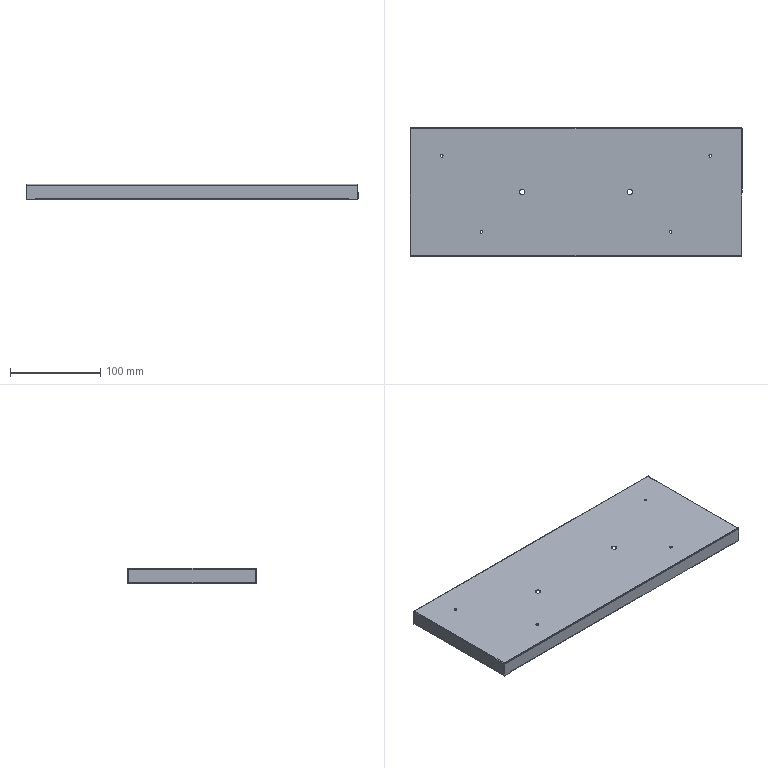Component | SolidWorks | DrawerWelding-1_DrawerPlate-1 | 1 solid | 94 faces | volume 76494 mm3 | plane 66 | cylinder 28 | commonest cylinder face diameters 3 x8 2.2 x8 0.2 x8 6 x4